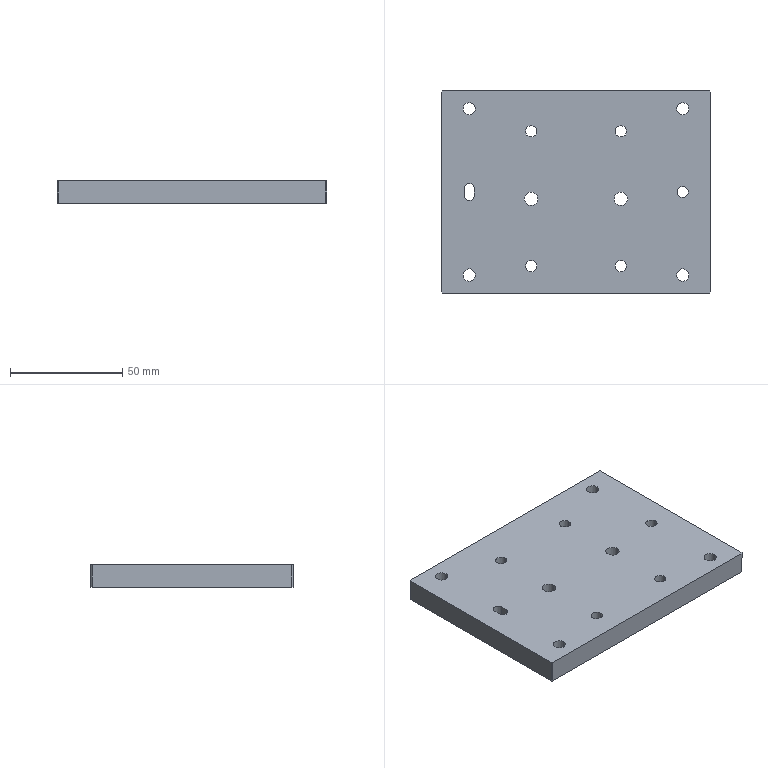Component | SolidWorks | 006-1 | 1 solid | 48 faces | box 120 x 90 x 10 mm | volume 103959 mm3 | cylinder 32 | plane 16 | commonest cylinder face diameters 5 x10 10 x8 5.5 x8 6 x4 4.45 x2 | material AL6061
build123d program:
from build123d import *

# Parameters (mm, degrees)
SKETCH1_W                                         = 120
SKETCH1_H                                         = 90
BOSS_EXTRUDE1_DEPTH                               = 10
CHAMFER1_SIZE                                     = 0.5
HOLE_SIZE_ACCORDING_TO_TYPE_OF_HEX_SO_D           = 5.5
HOLE_SIZE_ACCORDING_TO_TYPE_OF_HEX_SO_DEPTH       = 10.1
HOLE_SIZE_ACCORDING_TO_TYPE_OF_HEX_SO_CBORE_D     = 10
HOLE_SIZE_ACCORDING_TO_TYPE_OF_HEX_SO_CBORE_DEPTH = 5.7
HOLE_SIZE_ACCORDING_TO_TYPE_OF_HEX_SO_TIP         = 1.652
SKETCH6_R                                         = 2.5
CUT_EXTRUDE1_DEPTH                                = 76.664
M6_TAPPED_HOLE1_D                                 = 5
M6_TAPPED_HOLE1_DEPTH                             = 15
M6_TAPPED_HOLE1_TIP                               = 1.502
SIZE_MM_DOWEL_PIN_HOLE1_D                         = 6
SIZE_MM_DOWEL_PIN_HOLE1_DEPTH                     = 15
SIZE_MM_DOWEL_PIN_HOLE1_TIP                       = 1.803


with BuildPart() as part:
    # Sketch1 → Boss-Extrude1 (new body)
    with BuildSketch(Plane.XY):
        Rectangle(SKETCH1_W, SKETCH1_H)
    extrude(amount=BOSS_EXTRUDE1_DEPTH)

    # Chamfer1
    chamfer1_edges = [part.edges().sort_by_distance(p)[0] for p in [
        (60, -45, 5),
        (-60, -45, 5),
        (-60, 45, 5),
        (60, 45, 5),
    ]]
    chamfer(chamfer1_edges, length=CHAMFER1_SIZE)

    # Hole Size _ according to_ type of hex so
    with Locations(Plane.XY.offset(10)):
        with Locations((-47.5, 37), (47.5, -37), (47.5, 37), (-47.5, -37)):
            CounterBoreHole(HOLE_SIZE_ACCORDING_TO_TYPE_OF_HEX_SO_D / 2, HOLE_SIZE_ACCORDING_TO_TYPE_OF_HEX_SO_CBORE_D / 2, HOLE_SIZE_ACCORDING_TO_TYPE_OF_HEX_SO_CBORE_DEPTH, depth=HOLE_SIZE_ACCORDING_TO_TYPE_OF_HEX_SO_DEPTH)
            with Locations((0, 0, -(HOLE_SIZE_ACCORDING_TO_TYPE_OF_HEX_SO_DEPTH + HOLE_SIZE_ACCORDING_TO_TYPE_OF_HEX_SO_TIP / 2))):  # 118° drill point
                Cone(0, HOLE_SIZE_ACCORDING_TO_TYPE_OF_HEX_SO_D / 2, HOLE_SIZE_ACCORDING_TO_TYPE_OF_HEX_SO_TIP, mode=Mode.SUBTRACT)

    # Sketch6 → Cut-Extrude1 (cut, through all)
    with BuildSketch(Plane.XY.offset(10)):
        with Locations((-47.5, 0)):
            Circle(SKETCH6_R)
        with BuildLine():
            Line((45.275, -1.5), (45.275, 1.5))
            ThreePointArc((45.275, 1.5), (47.5, 3.725), (49.725, 1.5))
            Line((49.725, 1.5), (49.725, -1.5))
            ThreePointArc((49.725, -1.5), (47.5, -3.725), (45.275, -1.5))
        make_face()
    extrude(amount=-CUT_EXTRUDE1_DEPTH, mode=Mode.SUBTRACT)

    # M6 Tapped Hole1
    with Locations(Plane.XY.offset(10)):
        with Locations((-20, 27), (20, -33), (20, 27), (-20, -33)):
            Hole(M6_TAPPED_HOLE1_D / 2, depth=M6_TAPPED_HOLE1_DEPTH)
            with Locations((0, 0, -(M6_TAPPED_HOLE1_DEPTH + M6_TAPPED_HOLE1_TIP / 2))):  # 118° drill point
                Cone(0, M6_TAPPED_HOLE1_D / 2, M6_TAPPED_HOLE1_TIP, mode=Mode.SUBTRACT)

    # Size mm Dowel Pin Hole1
    with Locations(Plane.XY.offset(10)):
        with Locations((-20, -3), (20, -3)):
            Hole(SIZE_MM_DOWEL_PIN_HOLE1_D / 2, depth=SIZE_MM_DOWEL_PIN_HOLE1_DEPTH)
            with Locations((0, 0, -(SIZE_MM_DOWEL_PIN_HOLE1_DEPTH + SIZE_MM_DOWEL_PIN_HOLE1_TIP / 2))):  # 118° drill point
                Cone(0, SIZE_MM_DOWEL_PIN_HOLE1_D / 2, SIZE_MM_DOWEL_PIN_HOLE1_TIP, mode=Mode.SUBTRACT)


solid = part.part

# Placed as in the assembly
solid = solid.moved(Location((-240.455, -60.942, 154.696), (-180, 0, 180)))